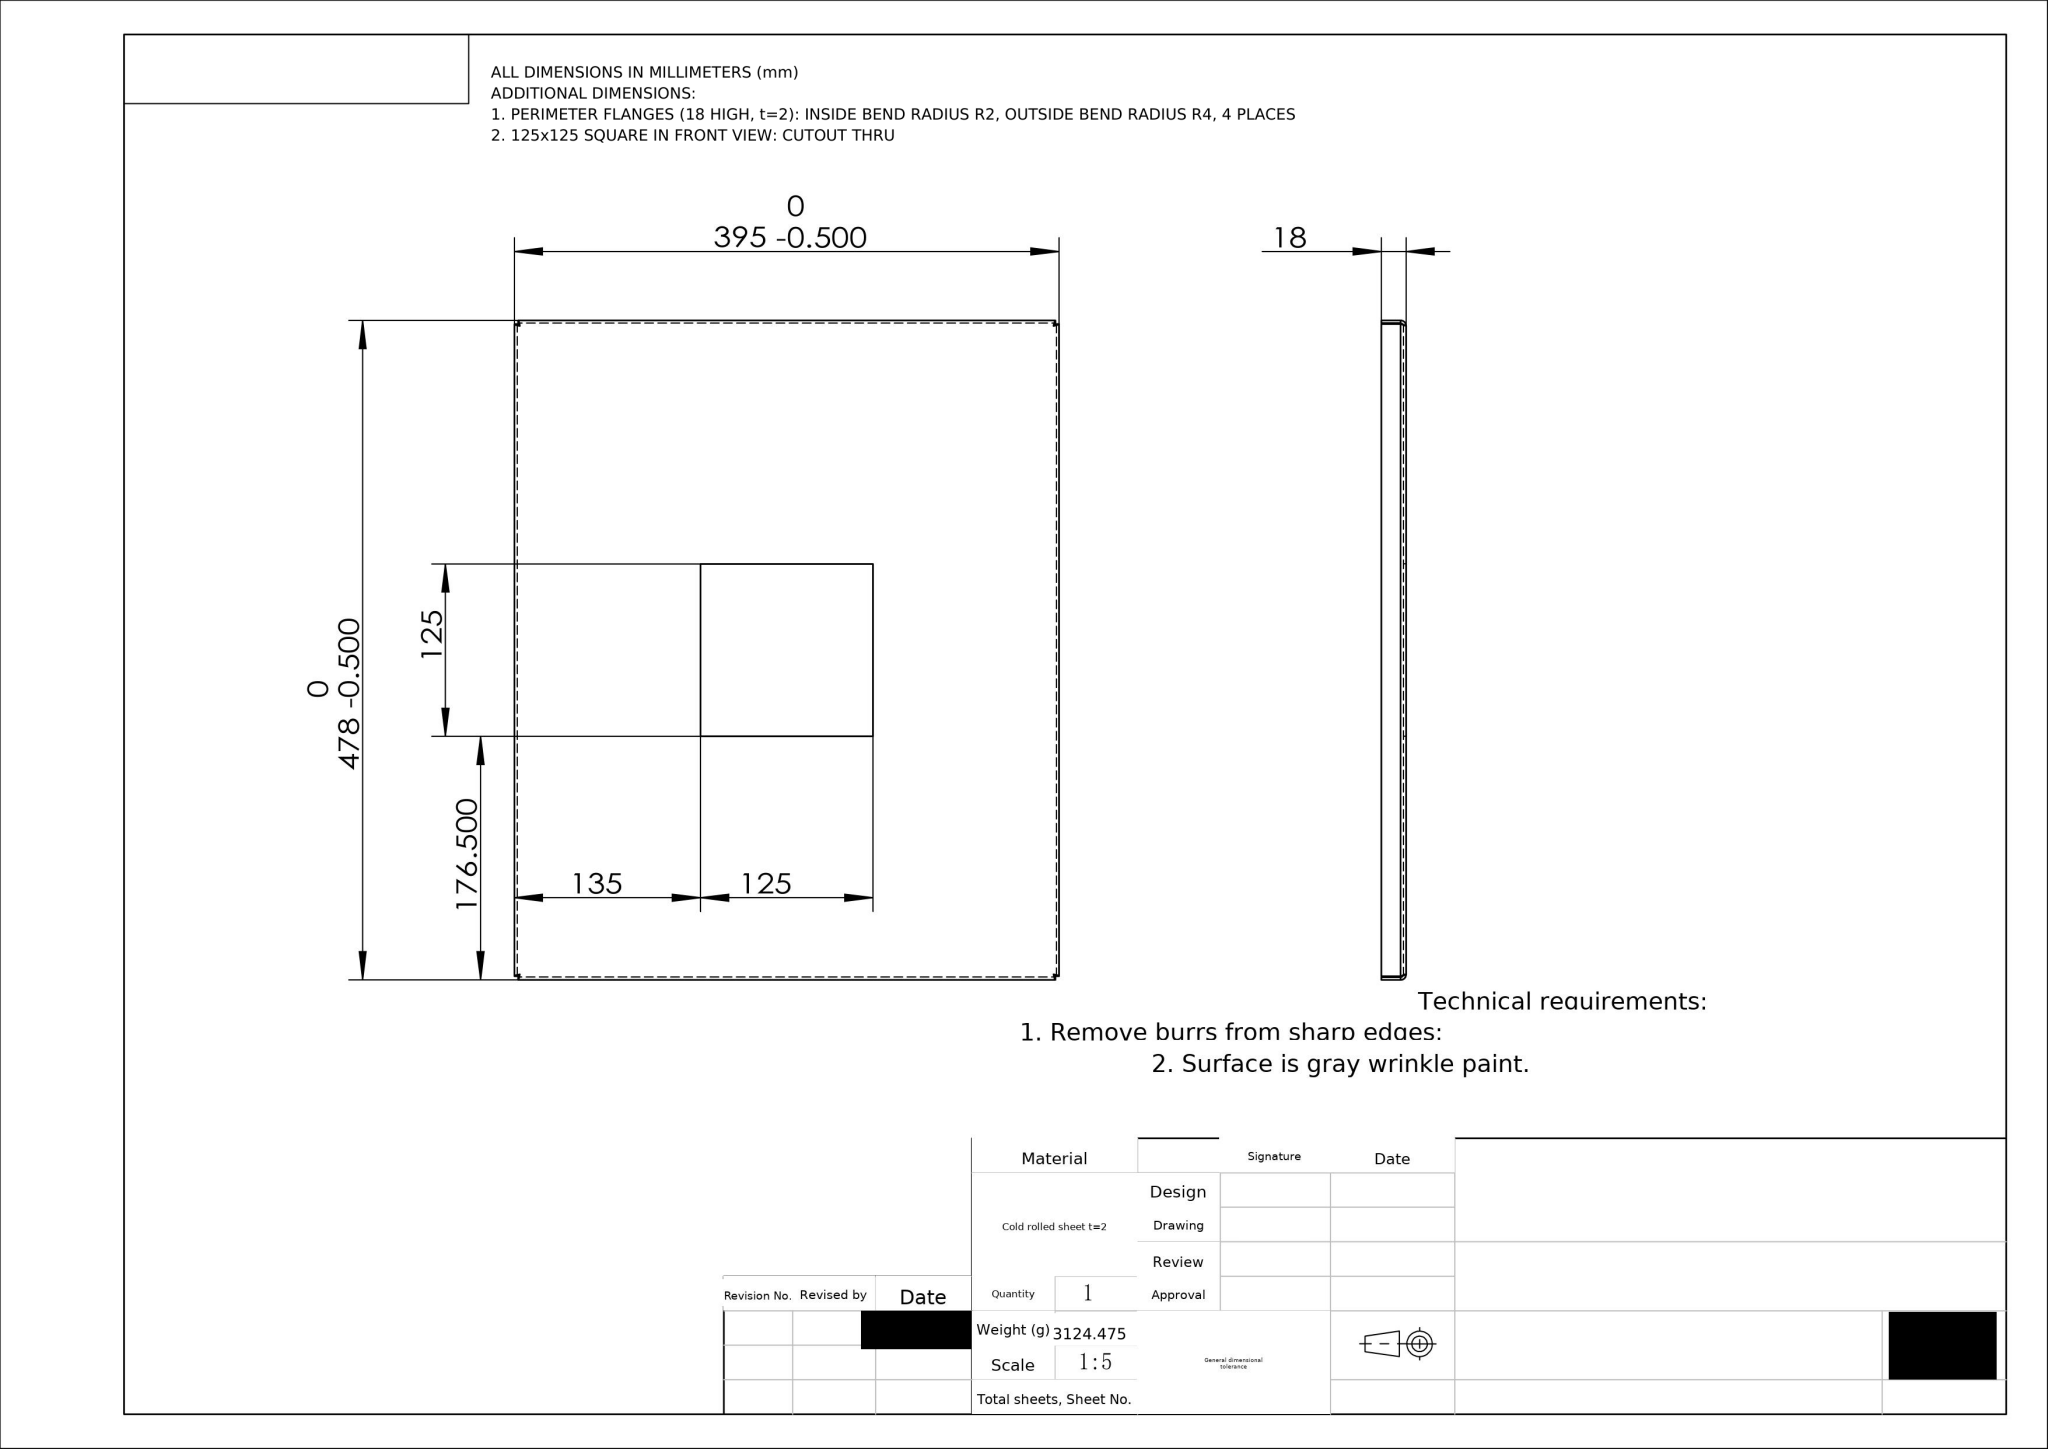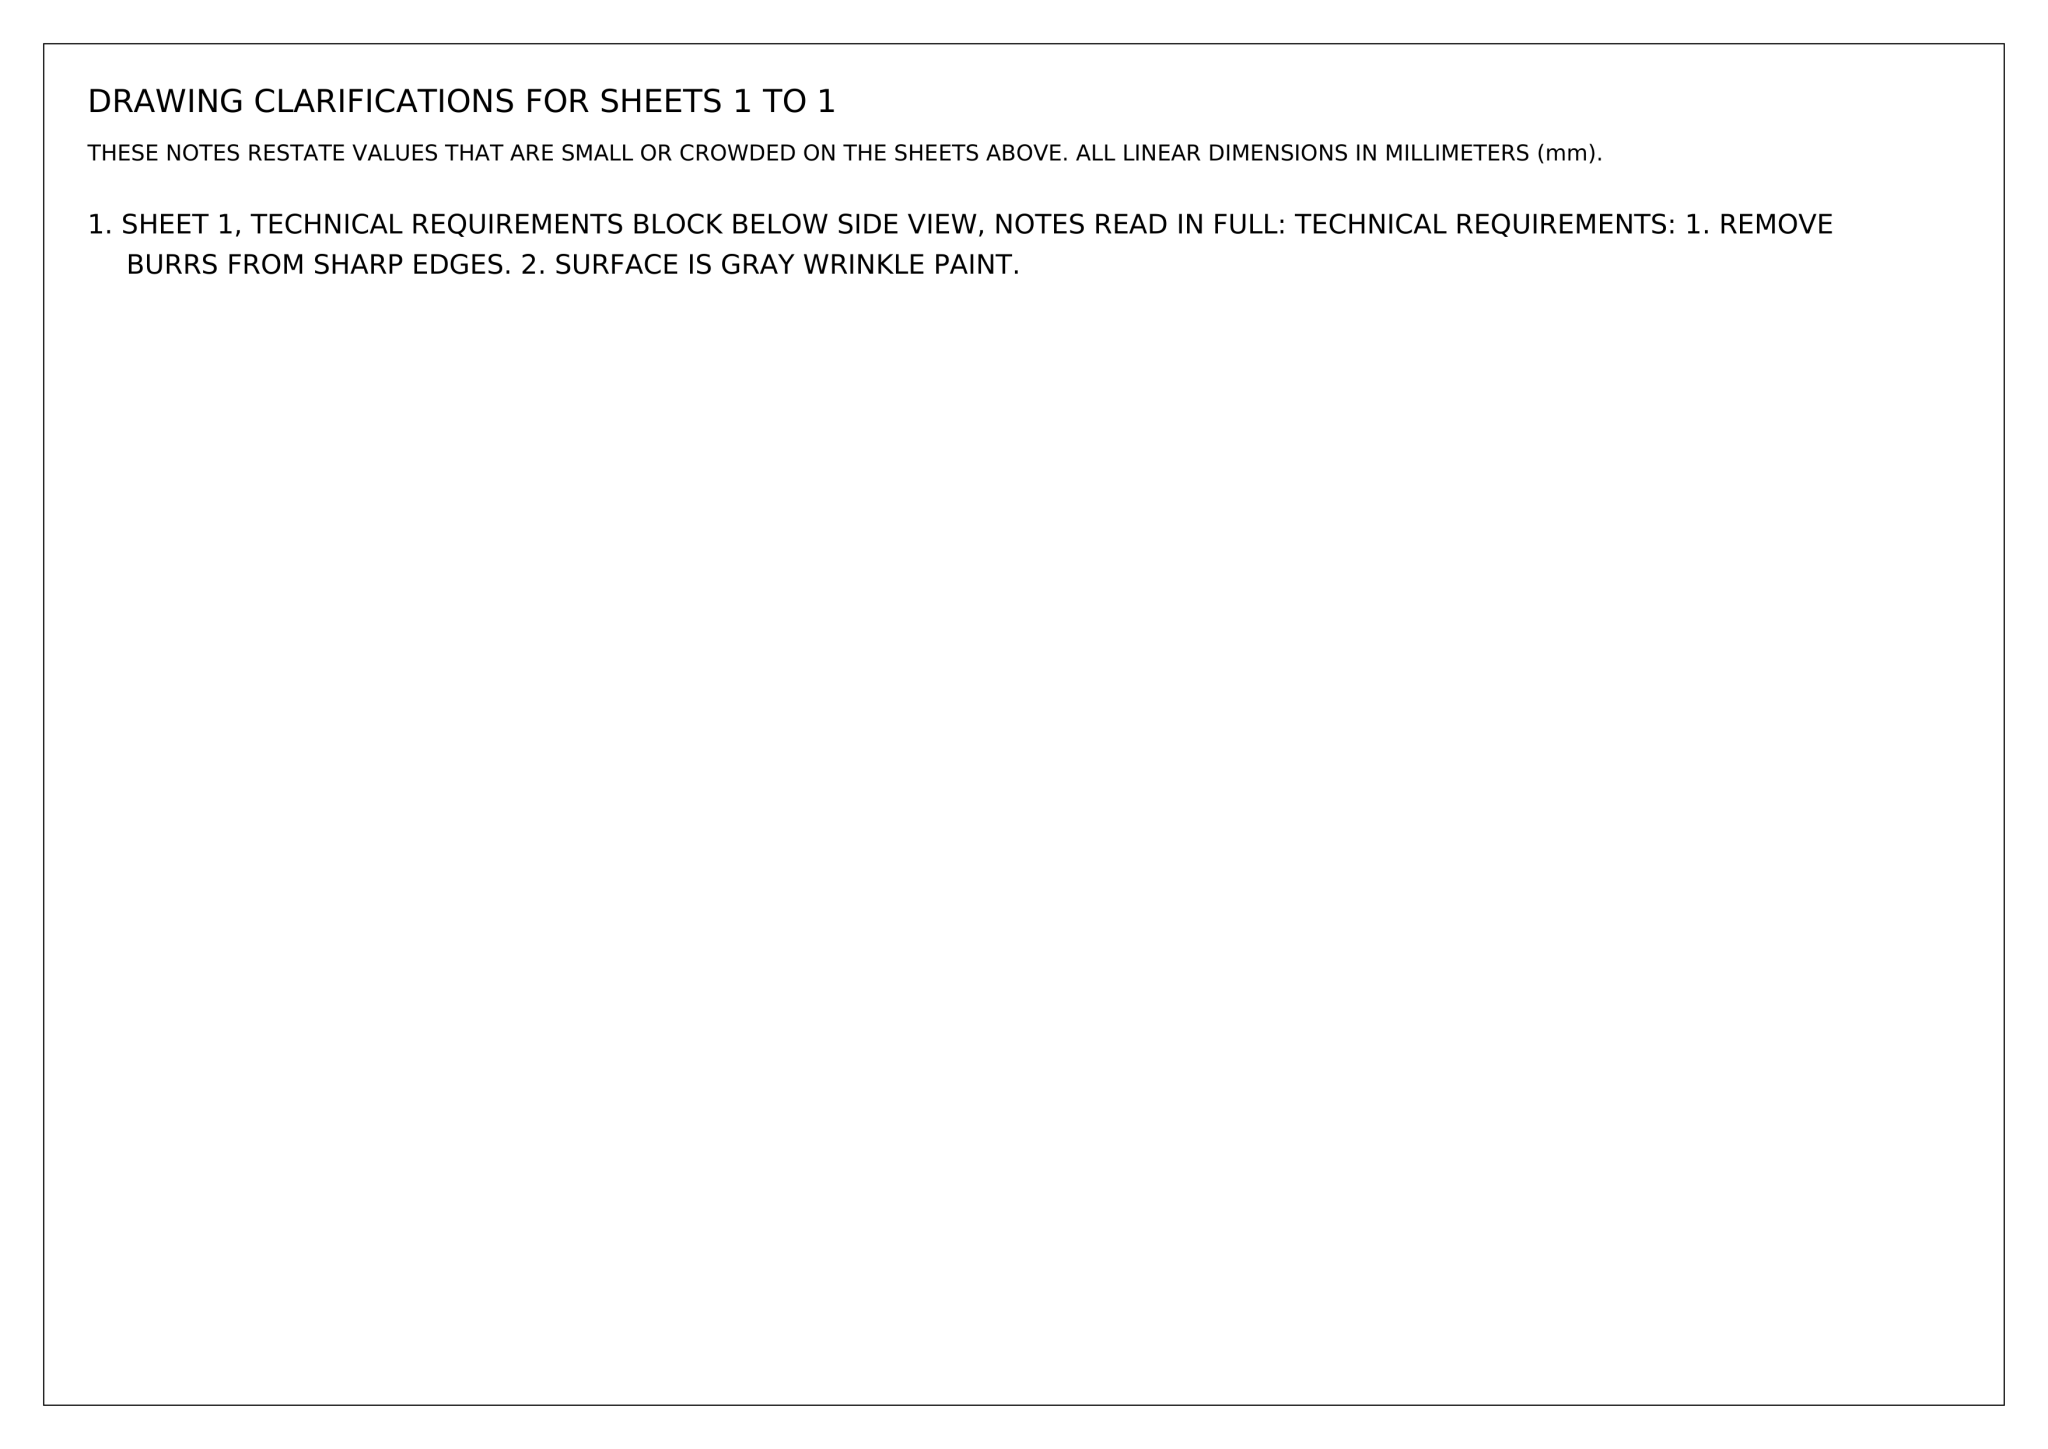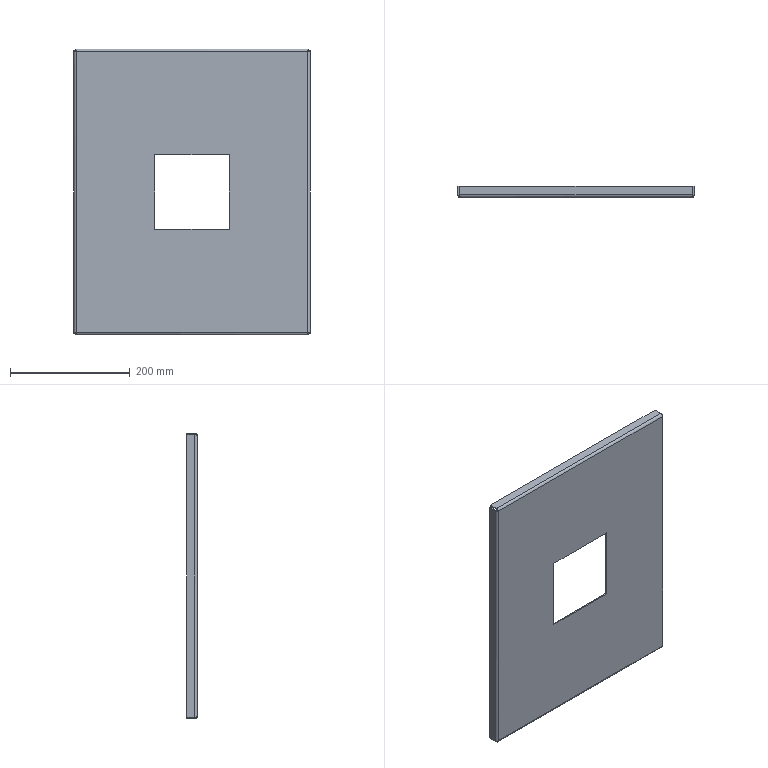Part | NX | mm | 1 solid | 42 faces | box 395 x 18 x 478 mm | volume 397014 mm3 | plane 26 | spline 8 | cylinder 8 | commonest cylinder face diameters 8 x4 4 x4